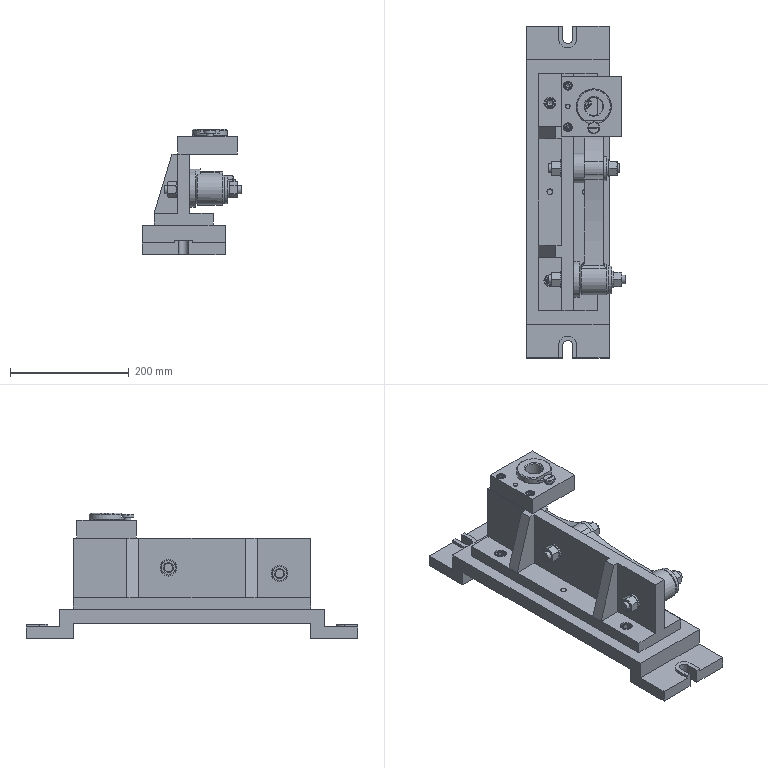Assembly | NX | mm | 28 component files | 28 solids | 509 faces | box 168 x 560 x 212 mm | volume 4365588 mm3 | plane 243 | cone 136 | cylinder 113 | torus 16 | spline 1 | commonest cylinder face diameters 4 x10 17 x8 14.376 x8 8 x7 42 x7 10 x6 20 x5 12 x5
Bill of materials:
GB-T6170_F-2000,M16x2 | 4 |  | Hexagonal prism with a central round through-bore; the corners are chamfered at both end faces. Looks like a hex nut.
unnamed part 1 | 1 |  | Long, slender link arm with a large cylindrical ring boss at one end, a smaller ring boss at the other end, and a through-hole in a widened section near the middle. A thin web joins the three, and a long recess or slot runs along its side.
unnamed part 2 | 1 |  | Flanged cylindrical bushing with a central through-bore. The flange is larger than the body and has chamfered edges. A partial-depth flat or notch is cut on one side of the flange.
GB-T119.1-2000,8x45 | 1 |  | Parallel Pin, GB-T 119.1-2000,8x45
unnamed part 3 | 1 |  | Square, thick block or plate with a large round through-hole placed off-centre. There are three smaller through-holes along one edge and one small hole with a conical bottom near another edge.
GB-T119.1-2000,10x35 | 2 |  | Parallel Pin, GB-T 119.1-2000,10x35
unnamed part 4 | 1 |  | Stepped cylindrical shaft: a short, larger-diameter central collar with small chamfered edges, and smaller-diameter pins sticking out on both sides at unequal lengths.
unnamed part 5 | 1 |  | Stepped, slotted-head pin. A cylindrical head with a chamfered top edge has a straight slot across its face. Below it are a shoulder of slightly smaller diameter, a reduced-diameter neck or groove, and an end pin with a chamfered tip.
unnamed part 6 | 1 |  | Flat circular disc with an open U-shaped slot running from the edge past the centre, ending in a round inner end. It forms a C-shaped slotted washer or plate.
GB-T848-2002,M16 | 4 |  | Thin flat annular ring (washer-like disc) with a single concentric circular through-hole and uniform thickness.
GB-T70.1-2000,M12x20 | 4 |  | Hexagon Socket Head Cap Screw, GB-T 70.1-2000,M12x20
unnamed part 7 | 1 |  | Flat circular disc with an open U-shaped slot running from the edge past the centre, ending in a round inner end. It forms a C-shaped slotted washer or plate.
unnamed part 8 | 1 |  | Short, thin-walled cylindrical ring or sleeve with a plain through-bore and small chamfers on the outer edges at both ends.
unnamed part 9 | 1 |  | Stepped cylindrical shaft: a larger-diameter central body with small chamfered edges, and smaller coaxial pins on both sides at unequal lengths.
unnamed part 10 | 1 |  | Long L-shaped bracket: a flat base plate with an upright wall whose back face slopes, so the wall tapers toward the top. Two cylindrical bosses with through-holes stand out from the front face of the wall. Small rectangular tabs are on the back, and several holes are in the base and along the top edge of the wall.
GB-T70.1-2000,M8x30 | 2 |  | Hexagon Socket Head Cap Screw, GB-T 70.1-2000,M8x30
unnamed part 11 | 1 |  | Long, flat, rectangular plate with an offset (joggled) profile: a raised central web and lower feet at each end, leaving a recess underneath. Each end has an open U-slot, and pairs of small holes run along the central web.
Mates:
1. fix | fixture_body 1 component
2. distance | BSMP3JX11L_3D 1 face | fixture_body 1 face
3. distance | BSMP3JX11L_3D 1 face | fixture_body 1 face
4. concentric | 42_locating_pin 1 edge | fixture_body 1 edge
5. concentric | 36_pad_block 1 edge | BSMP3JX11L_3D 1 edge
6. concentric | 46_pad_block 1 edge | BSMP3JX11L_3D 1 edge
7. concentric | GB-T848-2002_M16 3 edge | 36_pad_block 1 edge
8. concentric | GB-T6170_F-2000_M16x2 3 edge | GB-T848-2002_M16 3 edge
9. concentric | GB-T848-2002_M16 4 edge | 46_pad_block 1 edge
10. concentric | GB-T848-2002_M16 2 edge | fixture_body 1 edge
11. concentric | GB-T6170_F-2000_M16x2 1 edge | GB-T848-2002_M16 2 edge
12. concentric | GB-T848-2002_M16 1 edge | fixture_body 1 edge
13. concentric | GB-T6170_F-2000_M16x2 2 edge | GB-T848-2002_M16 1 edge
14. concentric | bushing 1 edge | boring_template 1 edge
15. concentric | boring_sleeve 1 edge | bushing 1 edge
16. touch align | boring_template 1 face | fixture_body 1 face
17. touch align | boring_sleeve 1 face | BSMP3JX11L_3D 1 face
18. touch align | boring_template 1 face | fixture_body 1 face
19. concentric | boring_sleeve_screw 1 edge | boring_template 1 arc
20. concentric | base_plate 1 arc | fixture_body 1 edge
21. concentric | 36_locating_pin 1 edge | fixture_body 1 edge
22. concentric | GB-T70_1-2000_M12x20 2 edge | fixture_body 1 edge
23. concentric | GB-T70_1-2000_M12x20 3 edge | fixture_body 1 edge
24. concentric | GB-T70_1-2000_M12x20 4 edge | fixture_body 1 edge
25. concentric | GB-T70_1-2000_M12x20 1 edge | fixture_body 1 edge
26. concentric | GB-T119_1-2000_10x35 1 edge | fixture_body 1 edge
27. concentric | GB-T119_1-2000_10x35 2 edge | fixture_body 1 edge
28. concentric | GB-T70_1-2000_M8x30 2 edge | boring_template 1 edge
29. concentric | GB-T70_1-2000_M8x30 1 edge | boring_template 1 edge
30. concentric | GB-T119_1-2000_8x45 1 edge | boring_template 1 edge
31. concentric | GB-T6170_F-2000_M16x2 4 edge | GB-T848-2002_M16 4 edge